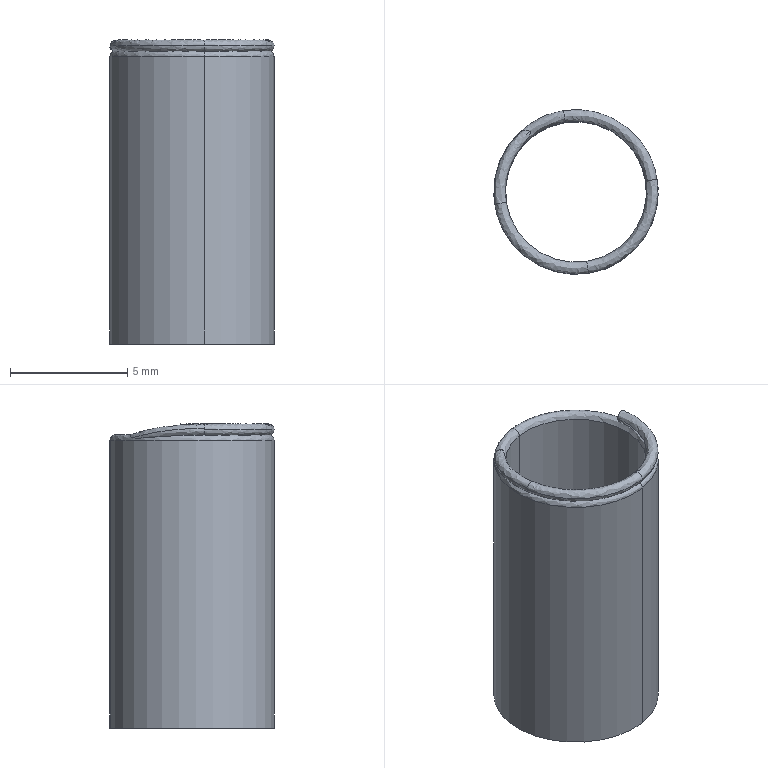Component | SolidWorks | SpringYIHEDAYVUR-D6-L15-1 | 1 solid | 18 faces | box 7 x 7 x 12.95 mm | volume 129 mm3 | spline 11 | cylinder 4 | plane 3 | commonest cylinder face diameters 7 x2 6 x2 | material 45
STEP:
#1=CARTESIAN_POINT('',(-0.4146,0.3527,-0.3228));
#2=VERTEX_POINT('',#1);
#3=CARTESIAN_POINT('',(-0.3728,0.08033,-0.3228));
#4=VERTEX_POINT('',#3);
#5=CARTESIAN_POINT('',(-0.3937,0.2165,-0.3228));
#6=DIRECTION('',(0.,0.,-1.));
#7=DIRECTION('',(-0.1516,0.9884,0.));
#8=AXIS2_PLACEMENT_3D('',#5,#6,#7);
#9=CIRCLE('',#8,0.1378);
#10=EDGE_CURVE('',#2,#4,#9,.T.);
#11=ORIENTED_EDGE('',*,*,#10,.F.);
#12=CARTESIAN_POINT('',(-0.4116,0.3333,-0.3228));
#13=VERTEX_POINT('',#12);
#14=CARTESIAN_POINT('',(-0.4131,0.343,-0.3228));
#15=DIRECTION('',(0.9884,0.1516,0.));
#16=DIRECTION('',(-0.1516,0.9884,0.));
#17=AXIS2_PLACEMENT_3D('',#14,#15,#16);
#18=CIRCLE('',#17,0.009843);
#19=EDGE_CURVE('',#2,#13,#18,.T.);
#20=ORIENTED_EDGE('',*,*,#19,.T.);
#21=CARTESIAN_POINT('',(-0.3758,0.09979,-0.3228));
#22=VERTEX_POINT('',#21);
#23=CARTESIAN_POINT('',(-0.3937,0.2165,-0.3228));
#24=DIRECTION('',(0.,0.,-1.));
#25=DIRECTION('',(0.1516,-0.9884,0.));
#26=AXIS2_PLACEMENT_3D('',#23,#24,#25);
#27=CIRCLE('',#26,0.1181);
#28=EDGE_CURVE('',#13,#22,#27,.T.);
#29=ORIENTED_EDGE('',*,*,#28,.T.);
#30=CARTESIAN_POINT('',(-0.3743,0.09006,-0.313));
#31=VERTEX_POINT('',#30);
#32=CARTESIAN_POINT('',(-0.3743,0.09006,-0.3228));
#33=DIRECTION('',(-0.9884,-0.1516,-0.));
#34=DIRECTION('',(0.1516,-0.9884,0.));
#35=AXIS2_PLACEMENT_3D('',#32,#33,#34);
#36=CIRCLE('',#35,0.009843);
#37=EDGE_CURVE('',#31,#22,#36,.T.);
#38=ORIENTED_EDGE('',*,*,#37,.F.);
#39=CARTESIAN_POINT('',(-0.2672,0.2359,-0.313));
#40=VERTEX_POINT('',#39);
#41=CARTESIAN_POINT('',(-0.3743,0.09006,-0.313));
#42=CARTESIAN_POINT('',(-0.3002,0.1014,-0.313));
#43=CARTESIAN_POINT('',(-0.2559,0.1618,-0.313));
#44=CARTESIAN_POINT('',(-0.2672,0.2359,-0.313));
#45=(BOUNDED_CURVE()B_SPLINE_CURVE(3,(#41,#42,#43,#44),.UNSPECIFIED.,.F.,.F.)B_SPLINE_CURVE_WITH_KNOTS((4,4),(0.6268,1.),.UNSPECIFIED.)CURVE()GEOMETRIC_REPRESENTATION_ITEM()RATIONAL_B_SPLINE_CURVE((1.,0.8047,0.8047,1.))REPRESENTATION_ITEM(''));
#46=EDGE_CURVE('',#31,#40,#45,.T.);
#47=ORIENTED_EDGE('',*,*,#46,.T.);
#48=CARTESIAN_POINT('',(-0.263,0.2366,-0.314));
#49=VERTEX_POINT('',#48);
#50=CARTESIAN_POINT('',(-0.2672,0.2359,-0.313));
#51=CARTESIAN_POINT('',(-0.2658,0.2362,-0.313));
#52=CARTESIAN_POINT('',(-0.2643,0.2364,-0.3133));
#53=CARTESIAN_POINT('',(-0.263,0.2366,-0.314));
#54=B_SPLINE_CURVE_WITH_KNOTS('',3,(#50,#51,#52,#53),.UNSPECIFIED.,.F.,.F.,(4,4),(0.,0.000112),.UNSPECIFIED.);
#55=EDGE_CURVE('',#40,#49,#54,.T.);
#56=ORIENTED_EDGE('',*,*,#55,.T.);
#57=CARTESIAN_POINT('',(-0.3737,0.08582,-0.314));
#58=VERTEX_POINT('',#57);
#59=CARTESIAN_POINT('',(-0.3937,0.2165,-0.314));
#60=DIRECTION('',(0.,0.,-1.));
#61=DIRECTION('',(0.1516,-0.9884,0.));
#62=AXIS2_PLACEMENT_3D('',#59,#60,#61);
#63=CIRCLE('',#62,0.1322);
#64=EDGE_CURVE('',#49,#58,#63,.T.);
#65=ORIENTED_EDGE('',*,*,#64,.T.);
#66=CARTESIAN_POINT('',(-0.3743,0.09006,-0.3228));
#67=DIRECTION('',(-0.9884,-0.1516,-0.));
#68=DIRECTION('',(0.1516,-0.9884,0.));
#69=AXIS2_PLACEMENT_3D('',#66,#67,#68);
#70=CIRCLE('',#69,0.009843);
#71=EDGE_CURVE('',#4,#58,#70,.T.);
#72=ORIENTED_EDGE('',*,*,#71,.F.);
#73=EDGE_LOOP('',(#11,#20,#29,#38,#47,#56,#65,#72));
#74=FACE_OUTER_BOUND('',#73,.T.);
#75=CARTESIAN_POINT('',(-0.4146,0.3527,-0.3228));
#76=CARTESIAN_POINT('',(-0.1422,0.3945,-0.3228));
#77=CARTESIAN_POINT('',(-0.1004,0.1221,-0.3228));
#78=CARTESIAN_POINT('',(-0.3728,0.08033,-0.3228));
#79=CARTESIAN_POINT('',(-0.4146,0.3527,-0.3031));
#80=CARTESIAN_POINT('',(-0.1422,0.3945,-0.3031));
#81=CARTESIAN_POINT('',(-0.1004,0.1221,-0.3031));
#82=CARTESIAN_POINT('',(-0.3728,0.08033,-0.3031));
#83=CARTESIAN_POINT('',(-0.4116,0.3333,-0.3031));
#84=CARTESIAN_POINT('',(-0.1781,0.3691,-0.3031));
#85=CARTESIAN_POINT('',(-0.1423,0.1356,-0.3031));
#86=CARTESIAN_POINT('',(-0.3758,0.09979,-0.3031));
#87=CARTESIAN_POINT('',(-0.4116,0.3333,-0.3228));
#88=CARTESIAN_POINT('',(-0.1781,0.3691,-0.3228));
#89=CARTESIAN_POINT('',(-0.1423,0.1356,-0.3228));
#90=CARTESIAN_POINT('',(-0.3758,0.09979,-0.3228));
#91=(BOUNDED_SURFACE()B_SPLINE_SURFACE(3,3,((#75,#76,#77,#78),(#79,#80,#81,#82),(#83,#84,#85,#86),(#87,#88,#89,#90)),.UNSPECIFIED.,.F.,.F.,.F.)B_SPLINE_SURFACE_WITH_KNOTS((4,4),(4,4),(0.,1.),(0.,1.),.UNSPECIFIED.)GEOMETRIC_REPRESENTATION_ITEM()RATIONAL_B_SPLINE_SURFACE(((1.,0.3333,0.3333,1.),(0.3333,0.1111,0.1111,0.3333),(0.3333,0.1111,0.1111,0.3333),(1.,0.3333,0.3333,1.)))REPRESENTATION_ITEM('')SURFACE());
#92=ADVANCED_FACE('',(#74),#91,.T.);
#93=CARTESIAN_POINT('',(-0.3758,0.09979,-0.3051));
#94=VERTEX_POINT('',#93);
#95=CARTESIAN_POINT('',(-0.5104,0.1986,-0.3051));
#96=VERTEX_POINT('',#95);
#97=CARTESIAN_POINT('',(-0.3937,0.2165,-0.3051));
#98=DIRECTION('',(0.,0.,-1.));
#99=DIRECTION('',(0.1516,-0.9884,0.));
#100=AXIS2_PLACEMENT_3D('',#97,#98,#99);
#101=CIRCLE('',#100,0.1181);
#102=EDGE_CURVE('',#94,#96,#101,.T.);
#103=ORIENTED_EDGE('',*,*,#102,.F.);
#104=CARTESIAN_POINT('',(-0.3752,0.0959,-0.313));
#105=VERTEX_POINT('',#104);
#106=CARTESIAN_POINT('',(-0.3743,0.09006,-0.3051));
#107=DIRECTION('',(-0.9884,-0.1516,-0.));
#108=DIRECTION('',(0.1516,-0.9884,0.));
#109=AXIS2_PLACEMENT_3D('',#106,#107,#108);
#110=CIRCLE('',#109,0.009843);
#111=EDGE_CURVE('',#94,#105,#110,.T.);
#112=ORIENTED_EDGE('',*,*,#111,.T.);
#113=CARTESIAN_POINT('',(-0.5143,0.198,-0.313));
#114=VERTEX_POINT('',#113);
#115=CARTESIAN_POINT('',(-0.3937,0.2165,-0.313));
#116=DIRECTION('',(-0.,-0.,1.));
#117=DIRECTION('',(0.1516,-0.9884,0.));
#118=AXIS2_PLACEMENT_3D('',#115,#116,#117);
#119=CIRCLE('',#118,0.122);
#120=EDGE_CURVE('',#114,#105,#119,.T.);
#121=ORIENTED_EDGE('',*,*,#120,.F.);
#122=CARTESIAN_POINT('',(-0.5108,0.1986,-0.3077));
#123=VERTEX_POINT('',#122);
#124=CARTESIAN_POINT('',(-0.5202,0.1971,-0.3051));
#125=DIRECTION('',(-0.1516,0.9884,0.));
#126=DIRECTION('',(-0.9548,-0.1464,0.2588));
#127=AXIS2_PLACEMENT_3D('',#124,#125,#126);
#128=CIRCLE('',#127,0.009843);
#129=EDGE_CURVE('',#123,#114,#128,.T.);
#130=ORIENTED_EDGE('',*,*,#129,.F.);
#131=CARTESIAN_POINT('',(-0.5202,0.1971,-0.3051));
#132=DIRECTION('',(-0.1516,0.9884,0.));
#133=DIRECTION('',(-0.9548,-0.1464,0.2588));
#134=AXIS2_PLACEMENT_3D('',#131,#132,#133);
#135=CIRCLE('',#134,0.009843);
#136=EDGE_CURVE('',#96,#123,#135,.T.);
#137=ORIENTED_EDGE('',*,*,#136,.F.);
#138=EDGE_LOOP('',(#103,#112,#121,#130,#137));
#139=FACE_OUTER_BOUND('',#138,.T.);
#140=CARTESIAN_POINT('',(-0.3758,0.09979,-0.3051));
#141=CARTESIAN_POINT('',(-0.4442,0.0893,-0.3051));
#142=CARTESIAN_POINT('',(-0.5,0.1302,-0.3051));
#143=CARTESIAN_POINT('',(-0.5104,0.1986,-0.3051));
#144=CARTESIAN_POINT('',(-0.3758,0.09979,-0.3083));
#145=CARTESIAN_POINT('',(-0.4442,0.0893,-0.3083));
#146=CARTESIAN_POINT('',(-0.5,0.1302,-0.3083));
#147=CARTESIAN_POINT('',(-0.5104,0.1986,-0.3083));
#148=CARTESIAN_POINT('',(-0.3756,0.09839,-0.3111));
#149=CARTESIAN_POINT('',(-0.4448,0.08778,-0.3111));
#150=CARTESIAN_POINT('',(-0.5012,0.1292,-0.3111));
#151=CARTESIAN_POINT('',(-0.5118,0.1984,-0.3111));
#152=CARTESIAN_POINT('',(-0.3752,0.0959,-0.313));
#153=CARTESIAN_POINT('',(-0.4459,0.08506,-0.313));
#154=CARTESIAN_POINT('',(-0.5035,0.1274,-0.313));
#155=CARTESIAN_POINT('',(-0.5143,0.198,-0.313));
#156=(BOUNDED_SURFACE()B_SPLINE_SURFACE(3,3,((#140,#141,#142,#143),(#144,#145,#146,#147),(#148,#149,#150,#151),(#152,#153,#154,#155)),.UNSPECIFIED.,.F.,.F.,.F.)B_SPLINE_SURFACE_WITH_KNOTS((4,4),(4,4),(0.,1.),(0.,1.),.UNSPECIFIED.)GEOMETRIC_REPRESENTATION_ITEM()RATIONAL_B_SPLINE_SURFACE(((1.,0.8047,0.8047,1.),(0.9296,0.7481,0.7481,0.9296),(0.9296,0.7481,0.7481,0.9296),(1.,0.8047,0.8047,1.)))REPRESENTATION_ITEM('')SURFACE());
#157=ADVANCED_FACE('',(#139),#156,.T.);
#158=CARTESIAN_POINT('',(-0.5244,0.1965,-0.314));
#159=VERTEX_POINT('',#158);
#160=CARTESIAN_POINT('',(-0.3937,0.2165,-0.314));
#161=DIRECTION('',(0.,0.,-1.));
#162=DIRECTION('',(0.1516,-0.9884,0.));
#163=AXIS2_PLACEMENT_3D('',#160,#161,#162);
#164=CIRCLE('',#163,0.1322);
#165=EDGE_CURVE('',#58,#159,#164,.T.);
#166=ORIENTED_EDGE('',*,*,#165,.F.);
#167=CARTESIAN_POINT('',(-0.3728,0.08033,-0.3051));
#168=VERTEX_POINT('',#167);
#169=CARTESIAN_POINT('',(-0.3743,0.09006,-0.3051));
#170=DIRECTION('',(-0.9884,-0.1516,-0.));
#171=DIRECTION('',(0.1516,-0.9884,0.));
#172=AXIS2_PLACEMENT_3D('',#169,#170,#171);
#173=CIRCLE('',#172,0.009843);
#174=EDGE_CURVE('',#58,#168,#173,.T.);
#175=ORIENTED_EDGE('',*,*,#174,.T.);
#176=CARTESIAN_POINT('',(-0.5299,0.1957,-0.3051));
#177=VERTEX_POINT('',#176);
#178=CARTESIAN_POINT('',(-0.3937,0.2165,-0.3051));
#179=DIRECTION('',(0.,0.,-1.));
#180=DIRECTION('',(0.1516,-0.9884,0.));
#181=AXIS2_PLACEMENT_3D('',#178,#179,#180);
#182=CIRCLE('',#181,0.1378);
#183=EDGE_CURVE('',#168,#177,#182,.T.);
#184=ORIENTED_EDGE('',*,*,#183,.T.);
#185=CARTESIAN_POINT('',(-0.5202,0.1971,-0.3051));
#186=DIRECTION('',(-0.1516,0.9884,0.));
#187=DIRECTION('',(-0.9548,-0.1464,0.2588));
#188=AXIS2_PLACEMENT_3D('',#185,#186,#187);
#189=CIRCLE('',#188,0.009843);
#190=EDGE_CURVE('',#159,#177,#189,.T.);
#191=ORIENTED_EDGE('',*,*,#190,.F.);
#192=EDGE_LOOP('',(#166,#175,#184,#191));
#193=FACE_OUTER_BOUND('',#192,.T.);
#194=CARTESIAN_POINT('',(-0.3737,0.08582,-0.314));
#195=CARTESIAN_POINT('',(-0.4502,0.07408,-0.314));
#196=CARTESIAN_POINT('',(-0.5127,0.1199,-0.314));
#197=CARTESIAN_POINT('',(-0.5244,0.1965,-0.314));
#198=CARTESIAN_POINT('',(-0.3731,0.08237,-0.3123));
#199=CARTESIAN_POINT('',(-0.4517,0.07032,-0.3123));
#200=CARTESIAN_POINT('',(-0.5158,0.1174,-0.3123));
#201=CARTESIAN_POINT('',(-0.5279,0.196,-0.3123));
#202=CARTESIAN_POINT('',(-0.3728,0.08033,-0.309));
#203=CARTESIAN_POINT('',(-0.4526,0.0681,-0.309));
#204=CARTESIAN_POINT('',(-0.5177,0.1159,-0.309));
#205=CARTESIAN_POINT('',(-0.5299,0.1957,-0.309));
#206=CARTESIAN_POINT('',(-0.3728,0.08033,-0.3051));
#207=CARTESIAN_POINT('',(-0.4526,0.0681,-0.3051));
#208=CARTESIAN_POINT('',(-0.5177,0.1159,-0.3051));
#209=CARTESIAN_POINT('',(-0.5299,0.1957,-0.3051));
#210=(BOUNDED_SURFACE()B_SPLINE_SURFACE(3,3,((#194,#195,#196,#197),(#198,#199,#200,#201),(#202,#203,#204,#205),(#206,#207,#208,#209)),.UNSPECIFIED.,.F.,.F.,.F.)B_SPLINE_SURFACE_WITH_KNOTS((4,4),(4,4),(0.,1.),(0.,1.),.UNSPECIFIED.)GEOMETRIC_REPRESENTATION_ITEM()RATIONAL_B_SPLINE_SURFACE(((1.,0.8047,0.8047,1.),(0.8982,0.7228,0.7228,0.8982),(0.8982,0.7228,0.7228,0.8982),(1.,0.8047,0.8047,1.)))REPRESENTATION_ITEM('')SURFACE());
#211=ADVANCED_FACE('',(#193),#210,.T.);
#212=ORIENTED_EDGE('',*,*,#183,.F.);
#213=CARTESIAN_POINT('',(-0.3743,0.09006,-0.3051));
#214=DIRECTION('',(-0.9884,-0.1516,-0.));
#215=DIRECTION('',(0.1516,-0.9884,0.));
#216=AXIS2_PLACEMENT_3D('',#213,#214,#215);
#217=CIRCLE('',#216,0.009843);
#218=EDGE_CURVE('',#168,#94,#217,.T.);
#219=ORIENTED_EDGE('',*,*,#218,.T.);
#220=ORIENTED_EDGE('',*,*,#102,.T.);
#221=CARTESIAN_POINT('',(-0.5296,0.1957,-0.3026));
#222=VERTEX_POINT('',#221);
#223=CARTESIAN_POINT('',(-0.5202,0.1971,-0.3051));
#224=DIRECTION('',(-0.1516,0.9884,0.));
#225=DIRECTION('',(-0.9548,-0.1464,0.2588));
#226=AXIS2_PLACEMENT_3D('',#223,#224,#225);
#227=CIRCLE('',#226,0.009843);
#228=EDGE_CURVE('',#222,#96,#227,.T.);
#229=ORIENTED_EDGE('',*,*,#228,.F.);
#230=CARTESIAN_POINT('',(-0.5202,0.1971,-0.3051));
#231=DIRECTION('',(-0.1516,0.9884,0.));
#232=DIRECTION('',(-0.9548,-0.1464,0.2588));
#233=AXIS2_PLACEMENT_3D('',#230,#231,#232);
#234=CIRCLE('',#233,0.009843);
#235=EDGE_CURVE('',#177,#222,#234,.T.);
#236=ORIENTED_EDGE('',*,*,#235,.F.);
#237=EDGE_LOOP('',(#212,#219,#220,#229,#236));
#238=FACE_OUTER_BOUND('',#237,.T.);
#239=CARTESIAN_POINT('',(-0.3728,0.08033,-0.3051));
#240=CARTESIAN_POINT('',(-0.4526,0.0681,-0.3051));
#241=CARTESIAN_POINT('',(-0.5177,0.1159,-0.3051));
#242=CARTESIAN_POINT('',(-0.5299,0.1957,-0.3051));
#243=CARTESIAN_POINT('',(-0.3728,0.08033,-0.2854));
#244=CARTESIAN_POINT('',(-0.4526,0.0681,-0.2854));
#245=CARTESIAN_POINT('',(-0.5177,0.1159,-0.2854));
#246=CARTESIAN_POINT('',(-0.5299,0.1957,-0.2854));
#247=CARTESIAN_POINT('',(-0.3758,0.09979,-0.2854));
#248=CARTESIAN_POINT('',(-0.4442,0.0893,-0.2854));
#249=CARTESIAN_POINT('',(-0.5,0.1302,-0.2854));
#250=CARTESIAN_POINT('',(-0.5104,0.1986,-0.2854));
#251=CARTESIAN_POINT('',(-0.3758,0.09979,-0.3051));
#252=CARTESIAN_POINT('',(-0.4442,0.0893,-0.3051));
#253=CARTESIAN_POINT('',(-0.5,0.1302,-0.3051));
#254=CARTESIAN_POINT('',(-0.5104,0.1986,-0.3051));
#255=(BOUNDED_SURFACE()B_SPLINE_SURFACE(3,3,((#239,#240,#241,#242),(#243,#244,#245,#246),(#247,#248,#249,#250),(#251,#252,#253,#254)),.UNSPECIFIED.,.F.,.F.,.T.)B_SPLINE_SURFACE_WITH_KNOTS((4,4),(4,4),(0.,1.),(0.,1.),.UNSPECIFIED.)GEOMETRIC_REPRESENTATION_ITEM()RATIONAL_B_SPLINE_SURFACE(((1.,0.8047,0.8047,1.),(0.3333,0.2682,0.2682,0.3333),(0.3333,0.2682,0.2682,0.3333),(1.,0.8047,0.8047,1.)))REPRESENTATION_ITEM('')SURFACE());
#256=ADVANCED_FACE('',(#238),#255,.T.);
#257=CARTESIAN_POINT('',(-0.3728,0.08033,-0.805));
#258=VERTEX_POINT('',#257);
#259=CARTESIAN_POINT('',(-0.4146,0.3527,-0.805));
#260=VERTEX_POINT('',#259);
#261=CARTESIAN_POINT('',(-0.3937,0.2165,-0.805));
#262=DIRECTION('',(0.,0.,-1.));
#263=DIRECTION('',(-0.1516,0.9884,0.));
#264=AXIS2_PLACEMENT_3D('',#261,#262,#263);
#265=CIRCLE('',#264,0.1378);
#266=EDGE_CURVE('',#258,#260,#265,.T.);
#267=ORIENTED_EDGE('',*,*,#266,.F.);
#268=CARTESIAN_POINT('',(-0.3728,0.08033,-0.8642));
#269=DIRECTION('',(-0.,-0.,1.));
#270=VECTOR('',#269,39.37);
#271=LINE('',#268,#270);
#272=EDGE_CURVE('',#258,#4,#271,.T.);
#273=ORIENTED_EDGE('',*,*,#272,.T.);
#274=CARTESIAN_POINT('',(-0.3937,0.2165,-0.3228));
#275=DIRECTION('',(0.,0.,-1.));
#276=DIRECTION('',(-0.1516,0.9884,0.));
#277=AXIS2_PLACEMENT_3D('',#274,#275,#276);
#278=CIRCLE('',#277,0.1378);
#279=EDGE_CURVE('',#4,#2,#278,.T.);
#280=ORIENTED_EDGE('',*,*,#279,.T.);
#281=CARTESIAN_POINT('',(-0.4146,0.3527,-0.8642));
#282=DIRECTION('',(-0.,-0.,1.));
#283=VECTOR('',#282,39.37);
#284=LINE('',#281,#283);
#285=EDGE_CURVE('',#260,#2,#284,.T.);
#286=ORIENTED_EDGE('',*,*,#285,.F.);
#287=EDGE_LOOP('',(#267,#273,#280,#286));
#288=FACE_OUTER_BOUND('',#287,.T.);
#289=CARTESIAN_POINT('',(-0.3937,0.2165,-0.8642));
#290=DIRECTION('',(-0.,-0.,1.));
#291=DIRECTION('',(-0.1516,0.9884,0.));
#292=AXIS2_PLACEMENT_3D('',#289,#290,#291);
#293=CYLINDRICAL_SURFACE('',#292,0.1378);
#294=ADVANCED_FACE('',(#288),#293,.T.);
#295=ORIENTED_EDGE('',*,*,#136,.T.);
#296=CARTESIAN_POINT('',(-0.501,0.2661,-0.313));
#297=VERTEX_POINT('',#296);
#298=CARTESIAN_POINT('',(-0.4022,0.2152,-0.3371));
#299=DIRECTION('',(-0.2558,-0.03923,-0.9659));
#300=DIRECTION('',(-0.9548,-0.1464,0.2588));
#301=AXIS2_PLACEMENT_3D('',#298,#299,#300);
#302=CIRCLE('',#301,0.1138);
#303=EDGE_CURVE('',#123,#297,#302,.T.);
#304=ORIENTED_EDGE('',*,*,#303,.T.);
#305=CARTESIAN_POINT('',(-0.4717,0.318,-0.313));
#306=VERTEX_POINT('',#305);
#307=CARTESIAN_POINT('',(-0.4717,0.318,-0.313));
#308=CARTESIAN_POINT('',(-0.4711,0.3177,-0.313));
#309=CARTESIAN_POINT('',(-0.4706,0.3172,-0.313));
#310=CARTESIAN_POINT('',(-0.4701,0.316,-0.313));
#311=CARTESIAN_POINT('',(-0.4701,0.3153,-0.313));
#312=CARTESIAN_POINT('',(-0.4704,0.3134,-0.313));
#313=CARTESIAN_POINT('',(-0.471,0.3122,-0.313));
#314=CARTESIAN_POINT('',(-0.4727,0.3088,-0.313));
#315=CARTESIAN_POINT('',(-0.4742,0.3067,-0.313));
#316=CARTESIAN_POINT('',(-0.4786,0.3004,-0.313));
#317=CARTESIAN_POINT('',(-0.4817,0.2963,-0.313));
#318=CARTESIAN_POINT('',(-0.4907,0.2838,-0.313));
#319=CARTESIAN_POINT('',(-0.4963,0.2752,-0.313));
#320=CARTESIAN_POINT('',(-0.501,0.2661,-0.313));
#321=B_SPLINE_CURVE_WITH_KNOTS('',3,(#307,#308,#309,#310,#311,#312,#313,#314,#315,#316,#317,#318,#319,#320),.UNSPECIFIED.,.F.,.F.,(4,2,2,2,2,2,4),(0.,0.00004935,0.0000987,0.0001974,0.0003948,0.0007896,0.001579),.UNSPECIFIED.);
#322=EDGE_CURVE('',#306,#297,#321,.T.);
#323=ORIENTED_EDGE('',*,*,#322,.F.);
#324=CARTESIAN_POINT('',(-0.4876,0.316,-0.3186));
#325=VERTEX_POINT('',#324);
#326=CARTESIAN_POINT('',(-0.4876,0.316,-0.3186));
#327=CARTESIAN_POINT('',(-0.4864,0.317,-0.3183));
#328=CARTESIAN_POINT('',(-0.4852,0.3179,-0.318));
#329=CARTESIAN_POINT('',(-0.4827,0.3193,-0.317));
#330=CARTESIAN_POINT('',(-0.4814,0.3198,-0.3163));
#331=CARTESIAN_POINT('',(-0.4773,0.3203,-0.3143));
#332=CARTESIAN_POINT('',(-0.4745,0.3193,-0.313));
#333=CARTESIAN_POINT('',(-0.4717,0.318,-0.313));
#334=B_SPLINE_CURVE_WITH_KNOTS('',3,(#326,#327,#328,#329,#330,#331,#332,#333),.UNSPECIFIED.,.F.,.F.,(4,2,2,4),(0.00333,0.003446,0.003562,0.003794),.UNSPECIFIED.);
#335=EDGE_CURVE('',#325,#306,#334,.T.);
#336=ORIENTED_EDGE('',*,*,#335,.F.);
#337=CARTESIAN_POINT('',(-0.4022,0.2152,-0.3371));
#338=DIRECTION('',(-0.2558,-0.03923,-0.9659));
#339=DIRECTION('',(-0.9548,-0.1464,0.2588));
#340=AXIS2_PLACEMENT_3D('',#337,#338,#339);
#341=CIRCLE('',#340,0.1334);
#342=EDGE_CURVE('',#222,#325,#341,.T.);
#343=ORIENTED_EDGE('',*,*,#342,.F.);
#344=ORIENTED_EDGE('',*,*,#228,.T.);
#345=EDGE_LOOP('',(#295,#304,#323,#336,#343,#344));
#346=FACE_OUTER_BOUND('',#345,.T.);
#347=CARTESIAN_POINT('',(-0.5296,0.1957,-0.3026));
#348=CARTESIAN_POINT('',(-0.5374,0.247,-0.3026));
#349=CARTESIAN_POINT('',(-0.5181,0.2946,-0.3096));
#350=CARTESIAN_POINT('',(-0.4774,0.3244,-0.3216));
#351=CARTESIAN_POINT('',(-0.5245,0.1965,-0.2836));
#352=CARTESIAN_POINT('',(-0.5324,0.2477,-0.2836));
#353=CARTESIAN_POINT('',(-0.5131,0.2954,-0.2906));
#354=CARTESIAN_POINT('',(-0.4723,0.3251,-0.3026));
#355=CARTESIAN_POINT('',(-0.5057,0.1994,-0.2887));
#356=CARTESIAN_POINT('',(-0.5124,0.2431,-0.2887));
#357=CARTESIAN_POINT('',(-0.496,0.2837,-0.2947));
#358=CARTESIAN_POINT('',(-0.4613,0.309,-0.3049));
#359=CARTESIAN_POINT('',(-0.5108,0.1986,-0.3077));
#360=CARTESIAN_POINT('',(-0.5175,0.2423,-0.3077));
#361=CARTESIAN_POINT('',(-0.501,0.2829,-0.3137));
#362=CARTESIAN_POINT('',(-0.4663,0.3083,-0.3239));
#363=(BOUNDED_SURFACE()B_SPLINE_SURFACE(3,3,((#347,#348,#349,#350),(#351,#352,#353,#354),(#355,#356,#357,#358),(#359,#360,#361,#362)),.UNSPECIFIED.,.F.,.F.,.T.)B_SPLINE_SURFACE_WITH_KNOTS((4,4),(4,4),(0.,1.),(0.,1.),.UNSPECIFIED.)GEOMETRIC_REPRESENTATION_ITEM()RATIONAL_B_SPLINE_SURFACE(((1.,0.9007,0.9007,1.),(0.3333,0.3002,0.3002,0.3333),(0.3333,0.3002,0.3002,0.3333),(1.,0.9007,0.9007,1.)))REPRESENTATION_ITEM('')SURFACE());
#364=ADVANCED_FACE('',(#346),#363,.T.);
#365=ORIENTED_EDGE('',*,*,#235,.T.);
#366=ORIENTED_EDGE('',*,*,#342,.T.);
#367=CARTESIAN_POINT('',(-0.5244,0.1965,-0.314));
#368=CARTESIAN_POINT('',(-0.5261,0.2073,-0.314));
#369=CARTESIAN_POINT('',(-0.5268,0.2183,-0.3142));
#370=CARTESIAN_POINT('',(-0.5261,0.2346,-0.3147));
#371=CARTESIAN_POINT('',(-0.5255,0.2399,-0.3149));
#372=CARTESIAN_POINT('',(-0.5238,0.2507,-0.3154));
#373=CARTESIAN_POINT('',(-0.5226,0.256,-0.3157));
#374=CARTESIAN_POINT('',(-0.5181,0.2717,-0.3166));
#375=CARTESIAN_POINT('',(-0.5138,0.2815,-0.3174));
#376=CARTESIAN_POINT('',(-0.5055,0.2955,-0.3184));
#377=CARTESIAN_POINT('',(-0.5024,0.3,-0.3188));
#378=CARTESIAN_POINT('',(-0.4973,0.3064,-0.3191));
#379=CARTESIAN_POINT('',(-0.4955,0.3084,-0.3192));
#380=CARTESIAN_POINT('',(-0.4917,0.3124,-0.3191));
#381=CARTESIAN_POINT('',(-0.4897,0.3143,-0.319));
#382=CARTESIAN_POINT('',(-0.4876,0.316,-0.3186));
#383=B_SPLINE_CURVE_WITH_KNOTS('',3,(#367,#368,#369,#370,#371,#372,#373,#374,#375,#376,#377,#378,#379,#380,#381,#382),.UNSPECIFIED.,.F.,.F.,(4,2,2,2,2,2,2,4),(0.,0.0008326,0.001249,0.001665,0.002498,0.002914,0.003122,0.00333),.UNSPECIFIED.);
#384=EDGE_CURVE('',#159,#325,#383,.T.);
#385=ORIENTED_EDGE('',*,*,#384,.F.);
#386=ORIENTED_EDGE('',*,*,#190,.T.);
#387=EDGE_LOOP('',(#365,#366,#385,#386));
#388=FACE_OUTER_BOUND('',#387,.T.);
#389=CARTESIAN_POINT('',(-0.5243,0.1965,-0.314));
#390=CARTESIAN_POINT('',(-0.531,0.2401,-0.314));
#391=CARTESIAN_POINT('',(-0.5165,0.2814,-0.3195));
#392=CARTESIAN_POINT('',(-0.4844,0.3101,-0.3292));
#393=CARTESIAN_POINT('',(-0.5288,0.1958,-0.3119));
#394=CARTESIAN_POINT('',(-0.5357,0.2411,-0.3119));
#395=CARTESIAN_POINT('',(-0.5206,0.284,-0.3176));
#396=CARTESIAN_POINT('',(-0.4873,0.3138,-0.3277));
#397=CARTESIAN_POINT('',(-0.5308,0.1955,-0.3074));
#398=CARTESIAN_POINT('',(-0.538,0.2419,-0.3074));
#399=CARTESIAN_POINT('',(-0.5225,0.2859,-0.3133));
#400=CARTESIAN_POINT('',(-0.4883,0.3164,-0.3235));
#401=CARTESIAN_POINT('',(-0.5296,0.1957,-0.3026));
#402=CARTESIAN_POINT('',(-0.5367,0.2421,-0.3026));
#403=CARTESIAN_POINT('',(-0.5212,0.2861,-0.3085));
#404=CARTESIAN_POINT('',(-0.487,0.3166,-0.3187));
#405=(BOUNDED_SURFACE()B_SPLINE_SURFACE(3,3,((#389,#390,#391,#392),(#393,#394,#395,#396),(#397,#398,#399,#400),(#401,#402,#403,#404)),.UNSPECIFIED.,.F.,.F.,.F.)B_SPLINE_SURFACE_WITH_KNOTS((4,4),(4,4),(0.,1.),(0.,1.),.UNSPECIFIED.)GEOMETRIC_REPRESENTATION_ITEM()RATIONAL_B_SPLINE_SURFACE(((1.,0.9167,0.9167,1.),(0.8454,0.775,0.775,0.8454),(0.8454,0.775,0.775,0.8454),(1.,0.9167,0.9167,1.)))REPRESENTATION_ITEM('')SURFACE());
#406=ADVANCED_FACE('',(#388),#405,.T.);
#407=ORIENTED_EDGE('',*,*,#218,.F.);
#408=CARTESIAN_POINT('',(-0.2575,0.2374,-0.3051));
#409=VERTEX_POINT('',#408);
#410=CARTESIAN_POINT('',(-0.3937,0.2165,-0.3051));
#411=DIRECTION('',(0.,0.,-1.));
#412=DIRECTION('',(0.1516,-0.9884,0.));
#413=AXIS2_PLACEMENT_3D('',#410,#411,#412);
#414=CIRCLE('',#413,0.1378);
#415=EDGE_CURVE('',#409,#168,#414,.T.);
#416=ORIENTED_EDGE('',*,*,#415,.F.);
#417=CARTESIAN_POINT('',(-0.277,0.2344,-0.3051));
#418=VERTEX_POINT('',#417);
#419=CARTESIAN_POINT('',(-0.2575,0.2374,-0.3051));
#420=CARTESIAN_POINT('',(-0.2575,0.2374,-0.3025));
#421=CARTESIAN_POINT('',(-0.2586,0.2373,-0.3));
#422=CARTESIAN_POINT('',(-0.2621,0.2367,-0.2963));
#423=CARTESIAN_POINT('',(-0.2647,0.2363,-0.2953));
#424=CARTESIAN_POINT('',(-0.2698,0.2355,-0.2953));
#425=CARTESIAN_POINT('',(-0.2723,0.2351,-0.2963));
#426=CARTESIAN_POINT('',(-0.2759,0.2346,-0.3));
#427=CARTESIAN_POINT('',(-0.277,0.2344,-0.3026));
#428=CARTESIAN_POINT('',(-0.277,0.2344,-0.3051));
#429=B_SPLINE_CURVE_WITH_KNOTS('',3,(#419,#420,#421,#422,#423,#424,#425,#426,#427,#428),.UNSPECIFIED.,.F.,.F.,(4,2,2,2,4),(0.0002786,0.000474,0.0006694,0.0008649,0.00106),.UNSPECIFIED.);
#430=EDGE_CURVE('',#409,#418,#429,.T.);
#431=ORIENTED_EDGE('',*,*,#430,.T.);
#432=CARTESIAN_POINT('',(-0.3937,0.2165,-0.3051));
#433=DIRECTION('',(0.,0.,-1.));
#434=DIRECTION('',(0.1516,-0.9884,0.));
#435=AXIS2_PLACEMENT_3D('',#432,#433,#434);
#436=CIRCLE('',#435,0.1181);
#437=EDGE_CURVE('',#418,#94,#436,.T.);
#438=ORIENTED_EDGE('',*,*,#437,.T.);
#439=EDGE_LOOP('',(#407,#416,#431,#438));
#440=FACE_OUTER_BOUND('',#439,.T.);
#441=CARTESIAN_POINT('',(-0.2575,0.2374,-0.3051));
#442=CARTESIAN_POINT('',(-0.2453,0.1576,-0.3051));
#443=CARTESIAN_POINT('',(-0.293,0.09257,-0.3051));
#444=CARTESIAN_POINT('',(-0.3728,0.08033,-0.3051));
#445=CARTESIAN_POINT('',(-0.2575,0.2374,-0.2854));
#446=CARTESIAN_POINT('',(-0.2453,0.1576,-0.2854));
#447=CARTESIAN_POINT('',(-0.293,0.09257,-0.2854));
#448=CARTESIAN_POINT('',(-0.3728,0.08033,-0.2854));
#449=CARTESIAN_POINT('',(-0.277,0.2344,-0.2854));
#450=CARTESIAN_POINT('',(-0.2665,0.166,-0.2854));
#451=CARTESIAN_POINT('',(-0.3074,0.1103,-0.2854));
#452=CARTESIAN_POINT('',(-0.3758,0.09979,-0.2854));
#453=CARTESIAN_POINT('',(-0.277,0.2344,-0.3051));
#454=CARTESIAN_POINT('',(-0.2665,0.166,-0.3051));
#455=CARTESIAN_POINT('',(-0.3074,0.1103,-0.3051));
#456=CARTESIAN_POINT('',(-0.3758,0.09979,-0.3051));
#457=(BOUNDED_SURFACE()B_SPLINE_SURFACE(3,3,((#441,#442,#443,#444),(#445,#446,#447,#448),(#449,#450,#451,#452),(#453,#454,#455,#456)),.UNSPECIFIED.,.F.,.F.,.F.)B_SPLINE_SURFACE_WITH_KNOTS((4,4),(4,4),(0.,1.),(0.,1.),.UNSPECIFIED.)GEOMETRIC_REPRESENTATION_ITEM()RATIONAL_B_SPLINE_SURFACE(((1.,0.8047,0.8047,1.),(0.3333,0.2682,0.2682,0.3333),(0.3333,0.2682,0.2682,0.3333),(1.,0.8047,0.8047,1.)))REPRESENTATION_ITEM('')SURFACE());
#458=ADVANCED_FACE('',(#440),#457,.T.);
#459=ORIENTED_EDGE('',*,*,#174,.F.);
#460=ORIENTED_EDGE('',*,*,#64,.F.);
#461=CARTESIAN_POINT('',(-0.263,0.2366,-0.314));
#462=CARTESIAN_POINT('',(-0.2597,0.2371,-0.3124));
#463=CARTESIAN_POINT('',(-0.2575,0.2374,-0.3088));
#464=CARTESIAN_POINT('',(-0.2575,0.2374,-0.3051));
#465=B_SPLINE_CURVE_WITH_KNOTS('',3,(#461,#462,#463,#464),.UNSPECIFIED.,.F.,.F.,(4,4),(0.,0.0002786),.UNSPECIFIED.);
#466=EDGE_CURVE('',#49,#409,#465,.T.);
#467=ORIENTED_EDGE('',*,*,#466,.T.);
#468=ORIENTED_EDGE('',*,*,#415,.T.);
#469=EDGE_LOOP('',(#459,#460,#467,#468));
#470=FACE_OUTER_BOUND('',#469,.T.);
#471=CARTESIAN_POINT('',(-0.263,0.2366,-0.314));
#472=CARTESIAN_POINT('',(-0.2512,0.16,-0.314));
#473=CARTESIAN_POINT('',(-0.2971,0.09756,-0.314));
#474=CARTESIAN_POINT('',(-0.3737,0.08582,-0.314));
#475=CARTESIAN_POINT('',(-0.2595,0.2371,-0.3123));
#476=CARTESIAN_POINT('',(-0.2475,0.1585,-0.3123));
#477=CARTESIAN_POINT('',(-0.2945,0.09442,-0.3123));
#478=CARTESIAN_POINT('',(-0.3731,0.08237,-0.3123));
#479=CARTESIAN_POINT('',(-0.2575,0.2374,-0.309));
#480=CARTESIAN_POINT('',(-0.2453,0.1576,-0.309));
#481=CARTESIAN_POINT('',(-0.293,0.09257,-0.309));
#482=CARTESIAN_POINT('',(-0.3728,0.08033,-0.309));
#483=CARTESIAN_POINT('',(-0.2575,0.2374,-0.3051));
#484=CARTESIAN_POINT('',(-0.2453,0.1576,-0.3051));
#485=CARTESIAN_POINT('',(-0.293,0.09257,-0.3051));
#486=CARTESIAN_POINT('',(-0.3728,0.08033,-0.3051));
#487=(BOUNDED_SURFACE()B_SPLINE_SURFACE(3,3,((#471,#472,#473,#474),(#475,#476,#477,#478),(#479,#480,#481,#482),(#483,#484,#485,#486)),.UNSPECIFIED.,.F.,.F.,.F.)B_SPLINE_SURFACE_WITH_KNOTS((4,4),(4,4),(0.,1.),(0.,1.),.UNSPECIFIED.)GEOMETRIC_REPRESENTATION_ITEM()RATIONAL_B_SPLINE_SURFACE(((1.,0.8047,0.8047,1.),(0.8982,0.7228,0.7228,0.8982),(0.8982,0.7228,0.7228,0.8982),(1.,0.8047,0.8047,1.)))REPRESENTATION_ITEM('')SURFACE());
#488=ADVANCED_FACE('',(#470),#487,.T.);
#489=CARTESIAN_POINT('',(-0.4116,0.3333,-0.805));
#490=VERTEX_POINT('',#489);
#491=CARTESIAN_POINT('',(-0.3758,0.09979,-0.805));
#492=VERTEX_POINT('',#491);
#493=CARTESIAN_POINT('',(-0.3937,0.2165,-0.805));
#494=DIRECTION('',(0.,0.,-1.));
#495=DIRECTION('',(-0.1516,0.9884,0.));
#496=AXIS2_PLACEMENT_3D('',#493,#494,#495);
#497=CIRCLE('',#496,0.1181);
#498=EDGE_CURVE('',#490,#492,#497,.T.);
#499=ORIENTED_EDGE('',*,*,#498,.T.);
#500=CARTESIAN_POINT('',(-0.3758,0.09979,-0.8642));
#501=DIRECTION('',(-0.,-0.,1.));
#502=VECTOR('',#501,39.37);
#503=LINE('',#500,#502);
#504=EDGE_CURVE('',#492,#22,#503,.T.);
#505=ORIENTED_EDGE('',*,*,#504,.T.);
#506=ORIENTED_EDGE('',*,*,#28,.F.);
#507=CARTESIAN_POINT('',(-0.4116,0.3333,-0.8642));
#508=DIRECTION('',(-0.,-0.,1.));
#509=VECTOR('',#508,39.37);
#510=LINE('',#507,#509);
#511=EDGE_CURVE('',#490,#13,#510,.T.);
#512=ORIENTED_EDGE('',*,*,#511,.F.);
#513=EDGE_LOOP('',(#499,#505,#506,#512));
#514=FACE_OUTER_BOUND('',#513,.T.);
#515=CARTESIAN_POINT('',(-0.3937,0.2165,-0.8642));
#516=DIRECTION('',(-0.,-0.,1.));
#517=DIRECTION('',(-0.1516,0.9884,0.));
#518=AXIS2_PLACEMENT_3D('',#515,#516,#517);
#519=CYLINDRICAL_SURFACE('',#518,0.1181);
#520=ADVANCED_FACE('',(#514),#519,.F.);
#521=ORIENTED_EDGE('',*,*,#272,.F.);
#522=CARTESIAN_POINT('',(-0.3937,0.2165,-0.805));
#523=DIRECTION('',(0.,0.,-1.));
#524=DIRECTION('',(-0.1516,0.9884,0.));
#525=AXIS2_PLACEMENT_3D('',#522,#523,#524);
#526=CIRCLE('',#525,0.1378);
#527=EDGE_CURVE('',#260,#258,#526,.T.);
#528=ORIENTED_EDGE('',*,*,#527,.F.);
#529=ORIENTED_EDGE('',*,*,#285,.T.);
#530=ORIENTED_EDGE('',*,*,#10,.T.);
#531=EDGE_LOOP('',(#521,#528,#529,#530));
#532=FACE_OUTER_BOUND('',#531,.T.);
#533=CARTESIAN_POINT('',(-0.3937,0.2165,-0.8642));
#534=DIRECTION('',(-0.,-0.,1.));
#535=DIRECTION('',(-0.1516,0.9884,0.));
#536=AXIS2_PLACEMENT_3D('',#533,#534,#535);
#537=CYLINDRICAL_SURFACE('',#536,0.1378);
#538=ADVANCED_FACE('',(#532),#537,.T.);
#539=ORIENTED_EDGE('',*,*,#19,.F.);
#540=ORIENTED_EDGE('',*,*,#279,.F.);
#541=ORIENTED_EDGE('',*,*,#71,.T.);
#542=ORIENTED_EDGE('',*,*,#165,.T.);
#543=ORIENTED_EDGE('',*,*,#384,.T.);
#544=ORIENTED_EDGE('',*,*,#335,.T.);
#545=CARTESIAN_POINT('',(-0.4717,0.318,-0.313));
#546=CARTESIAN_POINT('',(-0.6029,0.2171,-0.313));
#547=CARTESIAN_POINT('',(-0.5379,0.06498,-0.313));
#548=CARTESIAN_POINT('',(-0.3743,0.09006,-0.313));
#549=(BOUNDED_CURVE()B_SPLINE_CURVE(3,(#545,#546,#547,#548),.UNSPECIFIED.,.F.,.F.)B_SPLINE_CURVE_WITH_KNOTS((4,4),(0.,0.6268),.UNSPECIFIED.)CURVE()GEOMETRIC_REPRESENTATION_ITEM()RATIONAL_B_SPLINE_CURVE((1.,0.4993,0.4993,1.))REPRESENTATION_ITEM(''));
#550=EDGE_CURVE('',#306,#31,#549,.T.);
#551=ORIENTED_EDGE('',*,*,#550,.T.);
#552=ORIENTED_EDGE('',*,*,#37,.T.);
#553=CARTESIAN_POINT('',(-0.3937,0.2165,-0.3228));
#554=DIRECTION('',(0.,0.,-1.));
#555=DIRECTION('',(0.1516,-0.9884,0.));
#556=AXIS2_PLACEMENT_3D('',#553,#554,#555);
#557=CIRCLE('',#556,0.1181);
#558=EDGE_CURVE('',#22,#13,#557,.T.);
#559=ORIENTED_EDGE('',*,*,#558,.T.);
#560=EDGE_LOOP('',(#539,#540,#541,#542,#543,#544,#551,#552,#559));
#561=FACE_OUTER_BOUND('',#560,.T.);
#562=CARTESIAN_POINT('',(-0.3728,0.08033,-0.3228));
#563=CARTESIAN_POINT('',(-0.4526,0.0681,-0.3228));
#564=CARTESIAN_POINT('',(-0.5177,0.1159,-0.3228));
#565=CARTESIAN_POINT('',(-0.5299,0.1957,-0.3228));
#566=CARTESIAN_POINT('',(-0.5421,0.2754,-0.3228));
#567=CARTESIAN_POINT('',(-0.4944,0.3405,-0.3228));
#568=CARTESIAN_POINT('',(-0.4146,0.3527,-0.3228));
#569=CARTESIAN_POINT('',(-0.3728,0.08033,-0.3031));
#570=CARTESIAN_POINT('',(-0.4526,0.0681,-0.3031));
#571=CARTESIAN_POINT('',(-0.5177,0.1159,-0.3031));
#572=CARTESIAN_POINT('',(-0.5299,0.1957,-0.3031));
#573=CARTESIAN_POINT('',(-0.5421,0.2754,-0.3031));
#574=CARTESIAN_POINT('',(-0.4944,0.3405,-0.3031));
#575=CARTESIAN_POINT('',(-0.4146,0.3527,-0.3031));
#576=CARTESIAN_POINT('',(-0.3758,0.09979,-0.3031));
#577=CARTESIAN_POINT('',(-0.4442,0.0893,-0.3031));
#578=CARTESIAN_POINT('',(-0.5,0.1302,-0.3031));
#579=CARTESIAN_POINT('',(-0.5104,0.1986,-0.3031));
#580=CARTESIAN_POINT('',(-0.5209,0.267,-0.3031));
#581=CARTESIAN_POINT('',(-0.48,0.3228,-0.3031));
#582=CARTESIAN_POINT('',(-0.4116,0.3333,-0.3031));
#583=CARTESIAN_POINT('',(-0.3758,0.09979,-0.3228));
#584=CARTESIAN_POINT('',(-0.4442,0.0893,-0.3228));
#585=CARTESIAN_POINT('',(-0.5,0.1302,-0.3228));
#586=CARTESIAN_POINT('',(-0.5104,0.1986,-0.3228));
#587=CARTESIAN_POINT('',(-0.5209,0.267,-0.3228));
#588=CARTESIAN_POINT('',(-0.48,0.3228,-0.3228));
#589=CARTESIAN_POINT('',(-0.4116,0.3333,-0.3228));
#590=(BOUNDED_SURFACE()B_SPLINE_SURFACE(3,3,((#562,#563,#564,#565,#566,#567,#568),(#569,#570,#571,#572,#573,#574,#575),(#576,#577,#578,#579,#580,#581,#582),(#583,#584,#585,#586,#587,#588,#589)),.UNSPECIFIED.,.F.,.F.,.F.)B_SPLINE_SURFACE_WITH_KNOTS((4,4),(4,3,4),(0.,1.),(0.,0.5,1.),.UNSPECIFIED.)GEOMETRIC_REPRESENTATION_ITEM()RATIONAL_B_SPLINE_SURFACE(((1.,0.8047,0.8047,1.,0.8047,0.8047,1.),(0.3333,0.2682,0.2682,0.3333,0.2682,0.2682,0.3333),(0.3333,0.2682,0.2682,0.3333,0.2682,0.2682,0.3333),(1.,0.8047,0.8047,1.,0.8047,0.8047,1.)))REPRESENTATION_ITEM('')SURFACE());
#591=ADVANCED_FACE('',(#561),#590,.T.);
#592=CARTESIAN_POINT('',(-0.2731,0.235,-0.313));
#593=VERTEX_POINT('',#592);
#594=CARTESIAN_POINT('',(-0.2672,0.2359,-0.313));
#595=DIRECTION('',(0.9884,0.1516,0.));
#596=VECTOR('',#595,39.37);
#597=LINE('',#594,#596);
#598=EDGE_CURVE('',#593,#40,#597,.T.);
#599=ORIENTED_EDGE('',*,*,#598,.F.);
#600=CARTESIAN_POINT('',(-0.277,0.2344,-0.3051));
#601=CARTESIAN_POINT('',(-0.277,0.2344,-0.3081));
#602=CARTESIAN_POINT('',(-0.2755,0.2347,-0.3112));
#603=CARTESIAN_POINT('',(-0.2731,0.235,-0.313));
#604=B_SPLINE_CURVE_WITH_KNOTS('',3,(#600,#601,#602,#603),.UNSPECIFIED.,.F.,.F.,(4,4),(0.00106,0.001291),.UNSPECIFIED.);
#605=EDGE_CURVE('',#418,#593,#604,.T.);
#606=ORIENTED_EDGE('',*,*,#605,.F.);
#607=ORIENTED_EDGE('',*,*,#430,.F.);
#608=ORIENTED_EDGE('',*,*,#466,.F.);
#609=ORIENTED_EDGE('',*,*,#55,.F.);
#610=EDGE_LOOP('',(#599,#606,#607,#608,#609));
#611=FACE_OUTER_BOUND('',#610,.T.);
#612=CARTESIAN_POINT('',(-0.2672,0.2359,-0.3051));
#613=DIRECTION('',(0.1516,-0.9884,-0.));
#614=DIRECTION('',(0.9884,0.1516,0.));
#615=AXIS2_PLACEMENT_3D('',#612,#613,#614);
#616=PLANE('',#615);
#617=ADVANCED_FACE('',(#611),#616,.F.);
#618=ORIENTED_EDGE('',*,*,#322,.T.);
#619=CARTESIAN_POINT('',(-0.501,0.2661,-0.313));
#620=CARTESIAN_POINT('',(-0.5064,0.2556,-0.313));
#621=CARTESIAN_POINT('',(-0.5105,0.2447,-0.313));
#622=CARTESIAN_POINT('',(-0.5142,0.2275,-0.313));
#623=CARTESIAN_POINT('',(-0.515,0.2216,-0.313));
#624=CARTESIAN_POINT('',(-0.5155,0.2098,-0.313));
#625=CARTESIAN_POINT('',(-0.5152,0.2039,-0.313));
#626=CARTESIAN_POINT('',(-0.5143,0.198,-0.313));
#627=B_SPLINE_CURVE_WITH_KNOTS('',3,(#619,#620,#621,#622,#623,#624,#625,#626),.UNSPECIFIED.,.F.,.F.,(4,2,2,4),(0.001579,0.002488,0.002942,0.003397),.UNSPECIFIED.);
#628=EDGE_CURVE('',#297,#114,#627,.T.);
#629=ORIENTED_EDGE('',*,*,#628,.T.);
#630=ORIENTED_EDGE('',*,*,#120,.T.);
#631=CARTESIAN_POINT('',(-0.3937,0.2165,-0.313));
#632=DIRECTION('',(-0.,-0.,1.));
#633=DIRECTION('',(0.1516,-0.9884,0.));
#634=AXIS2_PLACEMENT_3D('',#631,#632,#633);
#635=CIRCLE('',#634,0.122);
#636=EDGE_CURVE('',#105,#593,#635,.T.);
#637=ORIENTED_EDGE('',*,*,#636,.T.);
#638=ORIENTED_EDGE('',*,*,#598,.T.);
#639=ORIENTED_EDGE('',*,*,#46,.F.);
#640=ORIENTED_EDGE('',*,*,#550,.F.);
#641=EDGE_LOOP('',(#618,#629,#630,#637,#638,#639,#640));
#642=FACE_OUTER_BOUND('',#641,.T.);
#643=CARTESIAN_POINT('',(-0.3937,0.2165,-0.313));
#644=DIRECTION('',(0.,0.,-1.));
#645=DIRECTION('',(0.1516,-0.9884,-0.));
#646=AXIS2_PLACEMENT_3D('',#643,#644,#645);
#647=PLANE('',#646);
#648=ADVANCED_FACE('',(#642),#647,.T.);
#649=ORIENTED_EDGE('',*,*,#303,.F.);
#650=ORIENTED_EDGE('',*,*,#129,.T.);
#651=ORIENTED_EDGE('',*,*,#628,.F.);
#652=EDGE_LOOP('',(#649,#650,#651));
#653=FACE_OUTER_BOUND('',#652,.T.);
#654=CARTESIAN_POINT('',(-0.5108,0.1986,-0.3077));
#655=CARTESIAN_POINT('',(-0.5144,0.222,-0.3077));
#656=CARTESIAN_POINT('',(-0.5109,0.2453,-0.3095));
#657=CARTESIAN_POINT('',(-0.5008,0.2665,-0.3131));
#658=CARTESIAN_POINT('',(-0.5114,0.1985,-0.3098));
#659=CARTESIAN_POINT('',(-0.5149,0.2219,-0.3098));
#660=CARTESIAN_POINT('',(-0.5115,0.2453,-0.3117));
#661=CARTESIAN_POINT('',(-0.5014,0.2664,-0.3152));
#662=CARTESIAN_POINT('',(-0.5126,0.1983,-0.3117));
#663=CARTESIAN_POINT('',(-0.5162,0.2219,-0.3117));
#664=CARTESIAN_POINT('',(-0.5128,0.2454,-0.3135));
#665=CARTESIAN_POINT('',(-0.5026,0.2666,-0.3171));
#666=CARTESIAN_POINT('',(-0.5144,0.198,-0.313));
#667=CARTESIAN_POINT('',(-0.518,0.2219,-0.313));
#668=CARTESIAN_POINT('',(-0.5145,0.2457,-0.3149));
#669=CARTESIAN_POINT('',(-0.5042,0.2672,-0.3185));
#670=(BOUNDED_SURFACE()B_SPLINE_SURFACE(3,3,((#654,#655,#656,#657),(#658,#659,#660,#661),(#662,#663,#664,#665),(#666,#667,#668,#669)),.UNSPECIFIED.,.F.,.F.,.T.)B_SPLINE_SURFACE_WITH_KNOTS((4,4),(4,4),(0.,1.),(0.,1.),.UNSPECIFIED.)GEOMETRIC_REPRESENTATION_ITEM()RATIONAL_B_SPLINE_SURFACE(((1.,0.9688,0.9688,1.),(0.963,0.9329,0.9329,0.963),(0.963,0.9329,0.9329,0.963),(1.,0.9688,0.9688,1.)))REPRESENTATION_ITEM('')SURFACE());
#671=ADVANCED_FACE('',(#653),#670,.T.);
#672=ORIENTED_EDGE('',*,*,#111,.F.);
#673=ORIENTED_EDGE('',*,*,#437,.F.);
#674=ORIENTED_EDGE('',*,*,#605,.T.);
#675=ORIENTED_EDGE('',*,*,#636,.F.);
#676=EDGE_LOOP('',(#672,#673,#674,#675));
#677=FACE_OUTER_BOUND('',#676,.T.);
#678=CARTESIAN_POINT('',(-0.277,0.2344,-0.3051));
#679=CARTESIAN_POINT('',(-0.2665,0.166,-0.3051));
#680=CARTESIAN_POINT('',(-0.3074,0.1103,-0.3051));
#681=CARTESIAN_POINT('',(-0.3758,0.09979,-0.3051));
#682=CARTESIAN_POINT('',(-0.277,0.2344,-0.3083));
#683=CARTESIAN_POINT('',(-0.2665,0.166,-0.3083));
#684=CARTESIAN_POINT('',(-0.3074,0.1103,-0.3083));
#685=CARTESIAN_POINT('',(-0.3758,0.09979,-0.3083));
#686=CARTESIAN_POINT('',(-0.2756,0.2347,-0.3111));
#687=CARTESIAN_POINT('',(-0.2649,0.1654,-0.3111));
#688=CARTESIAN_POINT('',(-0.3064,0.109,-0.3111));
#689=CARTESIAN_POINT('',(-0.3756,0.09839,-0.3111));
#690=CARTESIAN_POINT('',(-0.2731,0.235,-0.313));
#691=CARTESIAN_POINT('',(-0.2622,0.1644,-0.313));
#692=CARTESIAN_POINT('',(-0.3045,0.1067,-0.313));
#693=CARTESIAN_POINT('',(-0.3752,0.0959,-0.313));
#694=(BOUNDED_SURFACE()B_SPLINE_SURFACE(3,3,((#678,#679,#680,#681),(#682,#683,#684,#685),(#686,#687,#688,#689),(#690,#691,#692,#693)),.UNSPECIFIED.,.F.,.F.,.F.)B_SPLINE_SURFACE_WITH_KNOTS((4,4),(4,4),(0.,1.),(0.,1.),.UNSPECIFIED.)GEOMETRIC_REPRESENTATION_ITEM()RATIONAL_B_SPLINE_SURFACE(((1.,0.8047,0.8047,1.),(0.9296,0.7481,0.7481,0.9296),(0.9296,0.7481,0.7481,0.9296),(1.,0.8047,0.8047,1.)))REPRESENTATION_ITEM('')SURFACE());
#695=ADVANCED_FACE('',(#677),#694,.T.);
#696=ORIENTED_EDGE('',*,*,#504,.F.);
#697=CARTESIAN_POINT('',(-0.3937,0.2165,-0.805));
#698=DIRECTION('',(0.,0.,-1.));
#699=DIRECTION('',(-0.1516,0.9884,0.));
#700=AXIS2_PLACEMENT_3D('',#697,#698,#699);
#701=CIRCLE('',#700,0.1181);
#702=EDGE_CURVE('',#492,#490,#701,.T.);
#703=ORIENTED_EDGE('',*,*,#702,.T.);
#704=ORIENTED_EDGE('',*,*,#511,.T.);
#705=ORIENTED_EDGE('',*,*,#558,.F.);
#706=EDGE_LOOP('',(#696,#703,#704,#705));
#707=FACE_OUTER_BOUND('',#706,.T.);
#708=CARTESIAN_POINT('',(-0.3937,0.2165,-0.8642));
#709=DIRECTION('',(-0.,-0.,1.));
#710=DIRECTION('',(-0.1516,0.9884,0.));
#711=AXIS2_PLACEMENT_3D('',#708,#709,#710);
#712=CYLINDRICAL_SURFACE('',#711,0.1181);
#713=ADVANCED_FACE('',(#707),#712,.F.);
#714=ORIENTED_EDGE('',*,*,#527,.T.);
#715=ORIENTED_EDGE('',*,*,#266,.T.);
#716=EDGE_LOOP('',(#714,#715));
#717=FACE_OUTER_BOUND('',#716,.T.);
#718=ORIENTED_EDGE('',*,*,#498,.F.);
#719=ORIENTED_EDGE('',*,*,#702,.F.);
#720=EDGE_LOOP('',(#718,#719));
#721=FACE_BOUND('',#720,.T.);
#722=CARTESIAN_POINT('',(0.01635,0.1399,-0.805));
#723=DIRECTION('',(-0.,-0.,1.));
#724=DIRECTION('',(-0.1516,0.9884,0.));
#725=AXIS2_PLACEMENT_3D('',#722,#723,#724);
#726=PLANE('',#725);
#727=ADVANCED_FACE('',(#717,#721),#726,.F.);
#728=CLOSED_SHELL('',(#92,#157,#211,#256,#294,#364,#406,#458,#488,#520,#538,#591,#617,#648,#671,#695,#713,#727));
#729=MANIFOLD_SOLID_BREP('',#728);
#730=CARTESIAN_POINT('',(0.,0.,0.));
#731=DIRECTION('',(0.,0.,1.));
#732=DIRECTION('',(1.,0.,0.));
#733=AXIS2_PLACEMENT_3D('',#730,#731,#732);
#734=(LENGTH_UNIT()NAMED_UNIT(*)SI_UNIT($,.METRE.));
#735=LENGTH_MEASURE_WITH_UNIT(LENGTH_MEASURE(0.0254),#734);
#736=DIMENSIONAL_EXPONENTS(1.,0.,0.,0.,0.,0.,0.);
#737=(CONVERSION_BASED_UNIT('',#735)LENGTH_UNIT()NAMED_UNIT(#736));
#738=UNCERTAINTY_MEASURE_WITH_UNIT(LENGTH_MEASURE(0.00001),#737,'','');
#739=(NAMED_UNIT(*)PLANE_ANGLE_UNIT()SI_UNIT($,.RADIAN.));
#740=(NAMED_UNIT(*)SI_UNIT($,.STERADIAN.)SOLID_ANGLE_UNIT());
#741=(GEOMETRIC_REPRESENTATION_CONTEXT(3)GLOBAL_UNCERTAINTY_ASSIGNED_CONTEXT((#738))GLOBAL_UNIT_ASSIGNED_CONTEXT((#737,#739,#740))REPRESENTATION_CONTEXT('',''));
#742=ADVANCED_BREP_SHAPE_REPRESENTATION('',(#729,#733),#741);
#743=COLOUR_RGB('',0.7922,0.8196,0.9333);
#744=FILL_AREA_STYLE_COLOUR('',#743);
#745=FILL_AREA_STYLE('',(#744));
#746=SURFACE_STYLE_FILL_AREA(#745);
#747=SURFACE_SIDE_STYLE('',(#746));
#748=SURFACE_STYLE_USAGE(.BOTH.,#747);
#749=PRESENTATION_STYLE_ASSIGNMENT((#748));
#750=STYLED_ITEM('',(#749),#729);
#751=PRESENTATION_LAYER_ASSIGNMENT('','',(#750));
#752=(LENGTH_UNIT()NAMED_UNIT(*)SI_UNIT($,.METRE.));
#753=LENGTH_MEASURE_WITH_UNIT(LENGTH_MEASURE(0.0254),#752);
#754=DIMENSIONAL_EXPONENTS(1.,0.,0.,0.,0.,0.,0.);
#755=(CONVERSION_BASED_UNIT('',#753)LENGTH_UNIT()NAMED_UNIT(#754));
#756=UNCERTAINTY_MEASURE_WITH_UNIT(LENGTH_MEASURE(0.00001),#755,'','');
#757=(NAMED_UNIT(*)PLANE_ANGLE_UNIT()SI_UNIT($,.RADIAN.));
#758=(NAMED_UNIT(*)SI_UNIT($,.STERADIAN.)SOLID_ANGLE_UNIT());
#759=(GEOMETRIC_REPRESENTATION_CONTEXT(3)GLOBAL_UNCERTAINTY_ASSIGNED_CONTEXT((#756))GLOBAL_UNIT_ASSIGNED_CONTEXT((#755,#757,#758))REPRESENTATION_CONTEXT('',''));
#760=MECHANICAL_DESIGN_GEOMETRIC_PRESENTATION_REPRESENTATION('',(#750),#759);